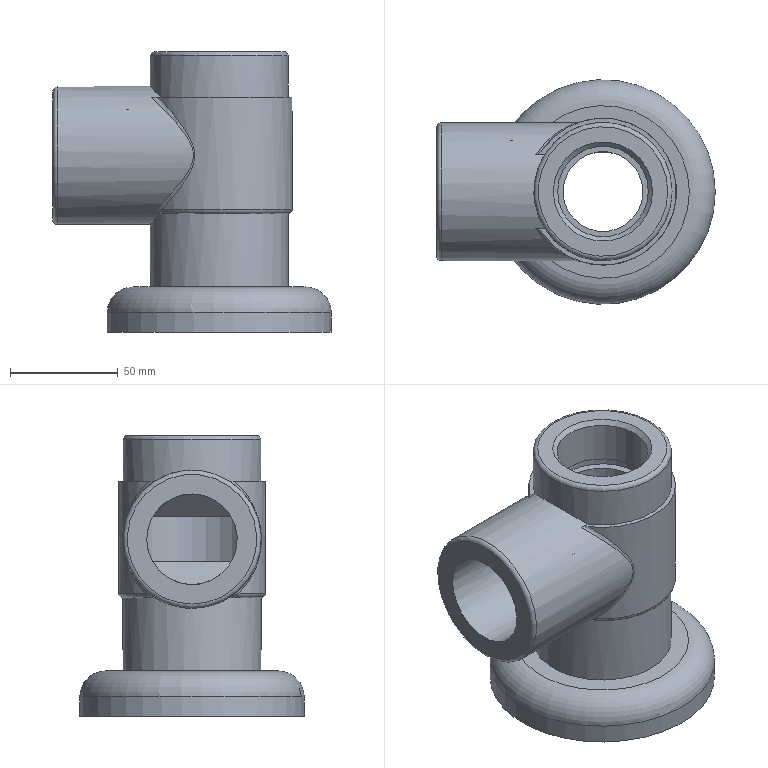Component | NX | VALVE_BODY | 1 solid | 61 faces | volume 371225 mm3 | plane 20 | cylinder 18 | cone 15 | spline 4 | torus 4 | commonest cylinder face diameters 7.9 x6 64 x3 42 x2 37 x1 104 x1 68 x1 44 x1 56 x1